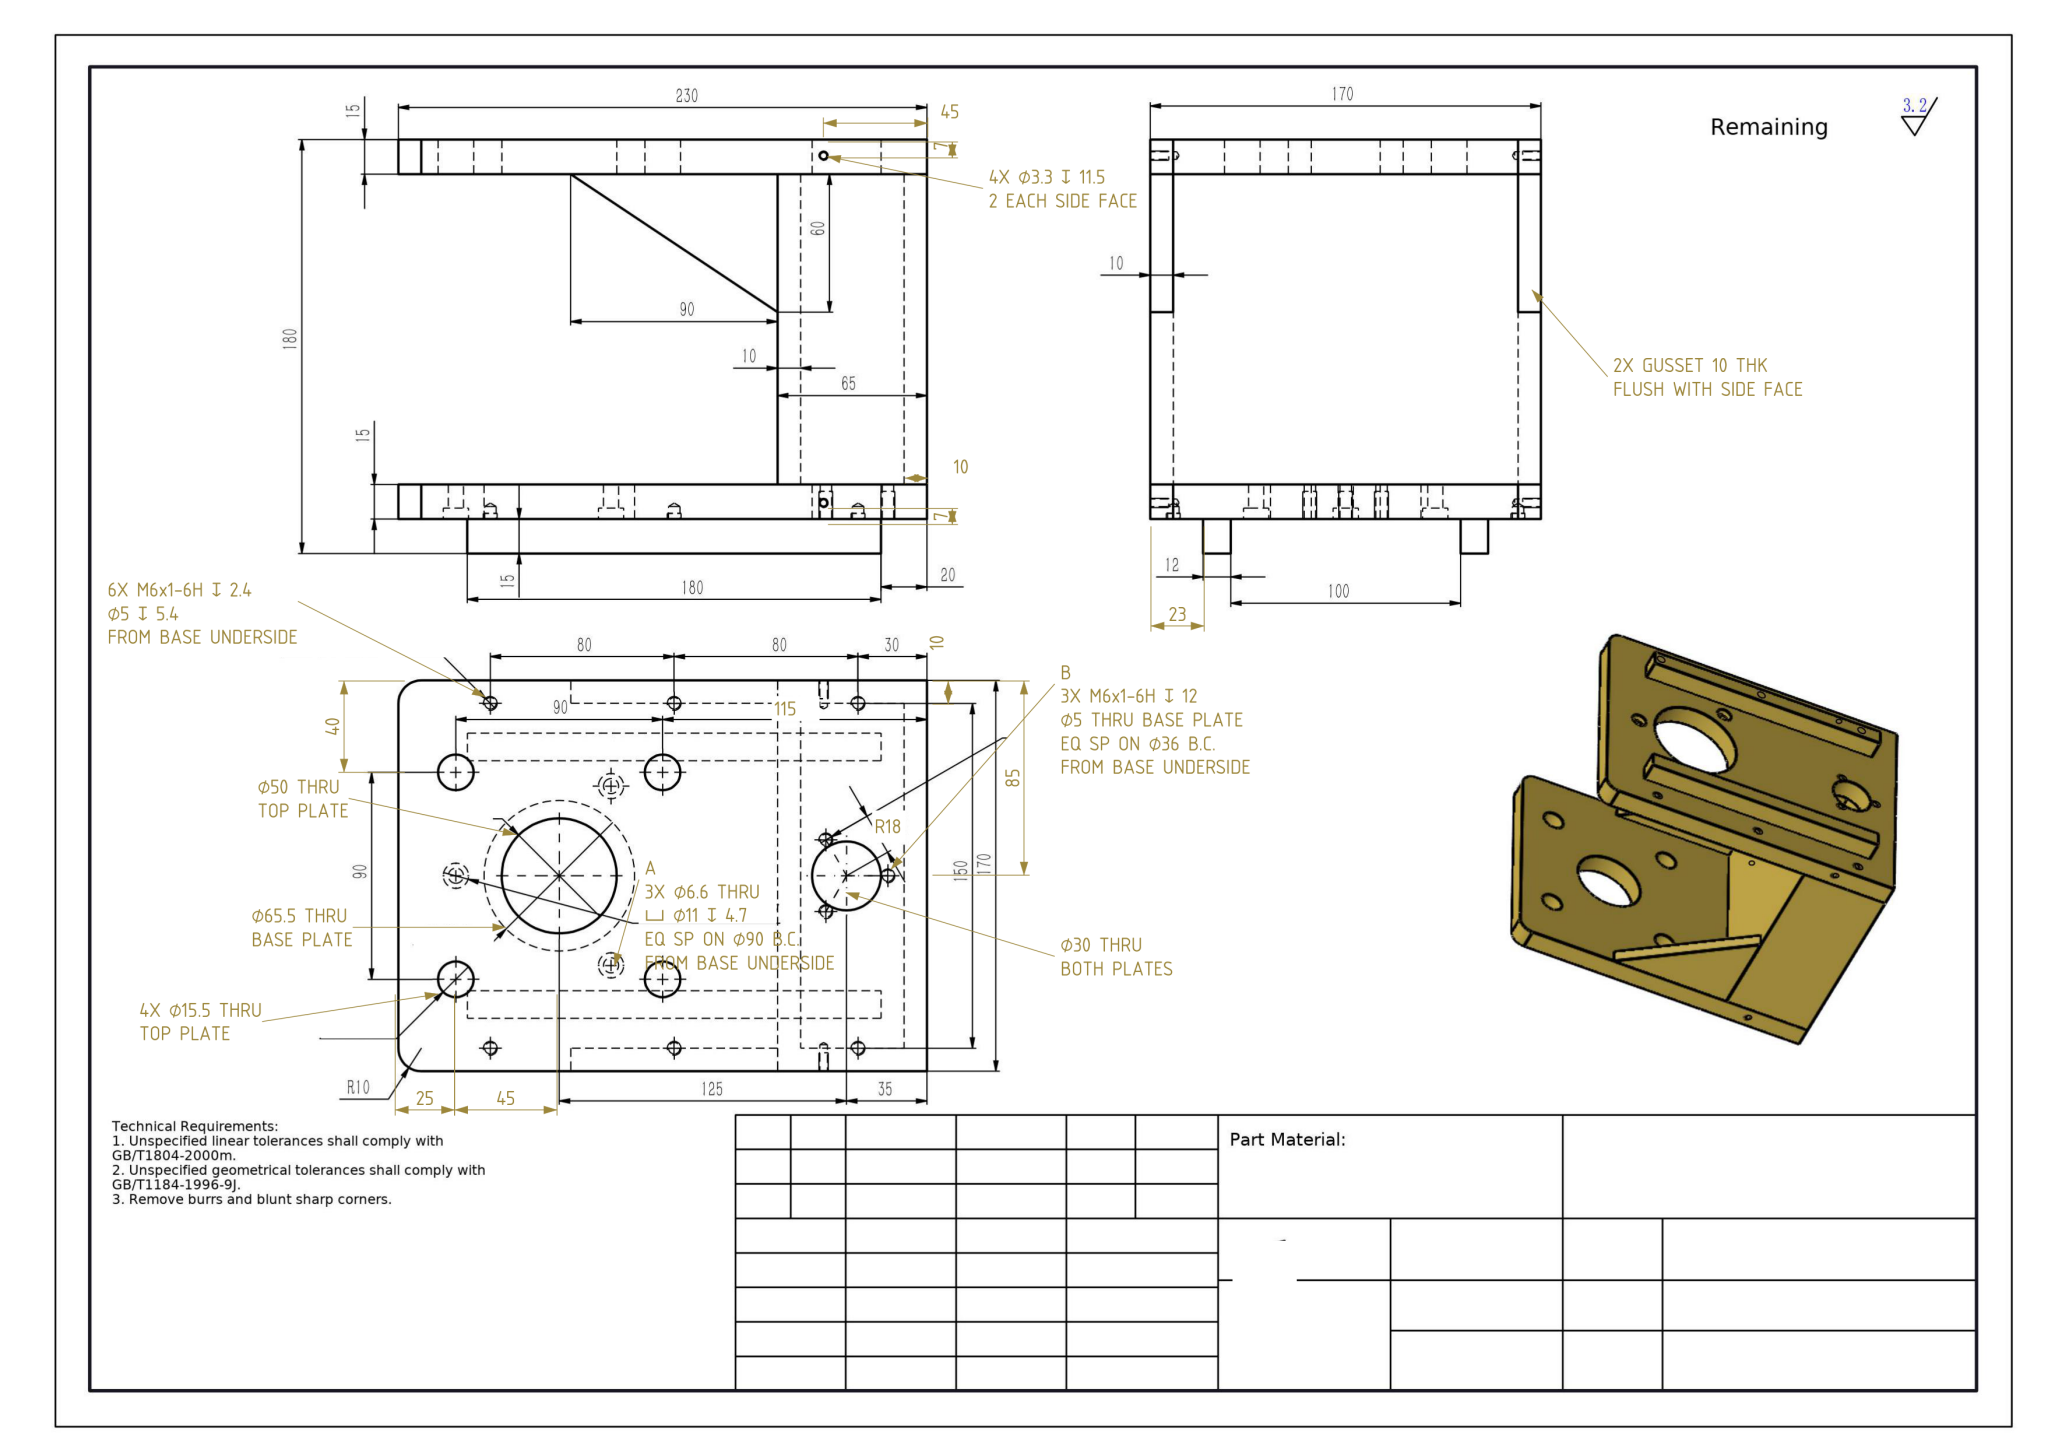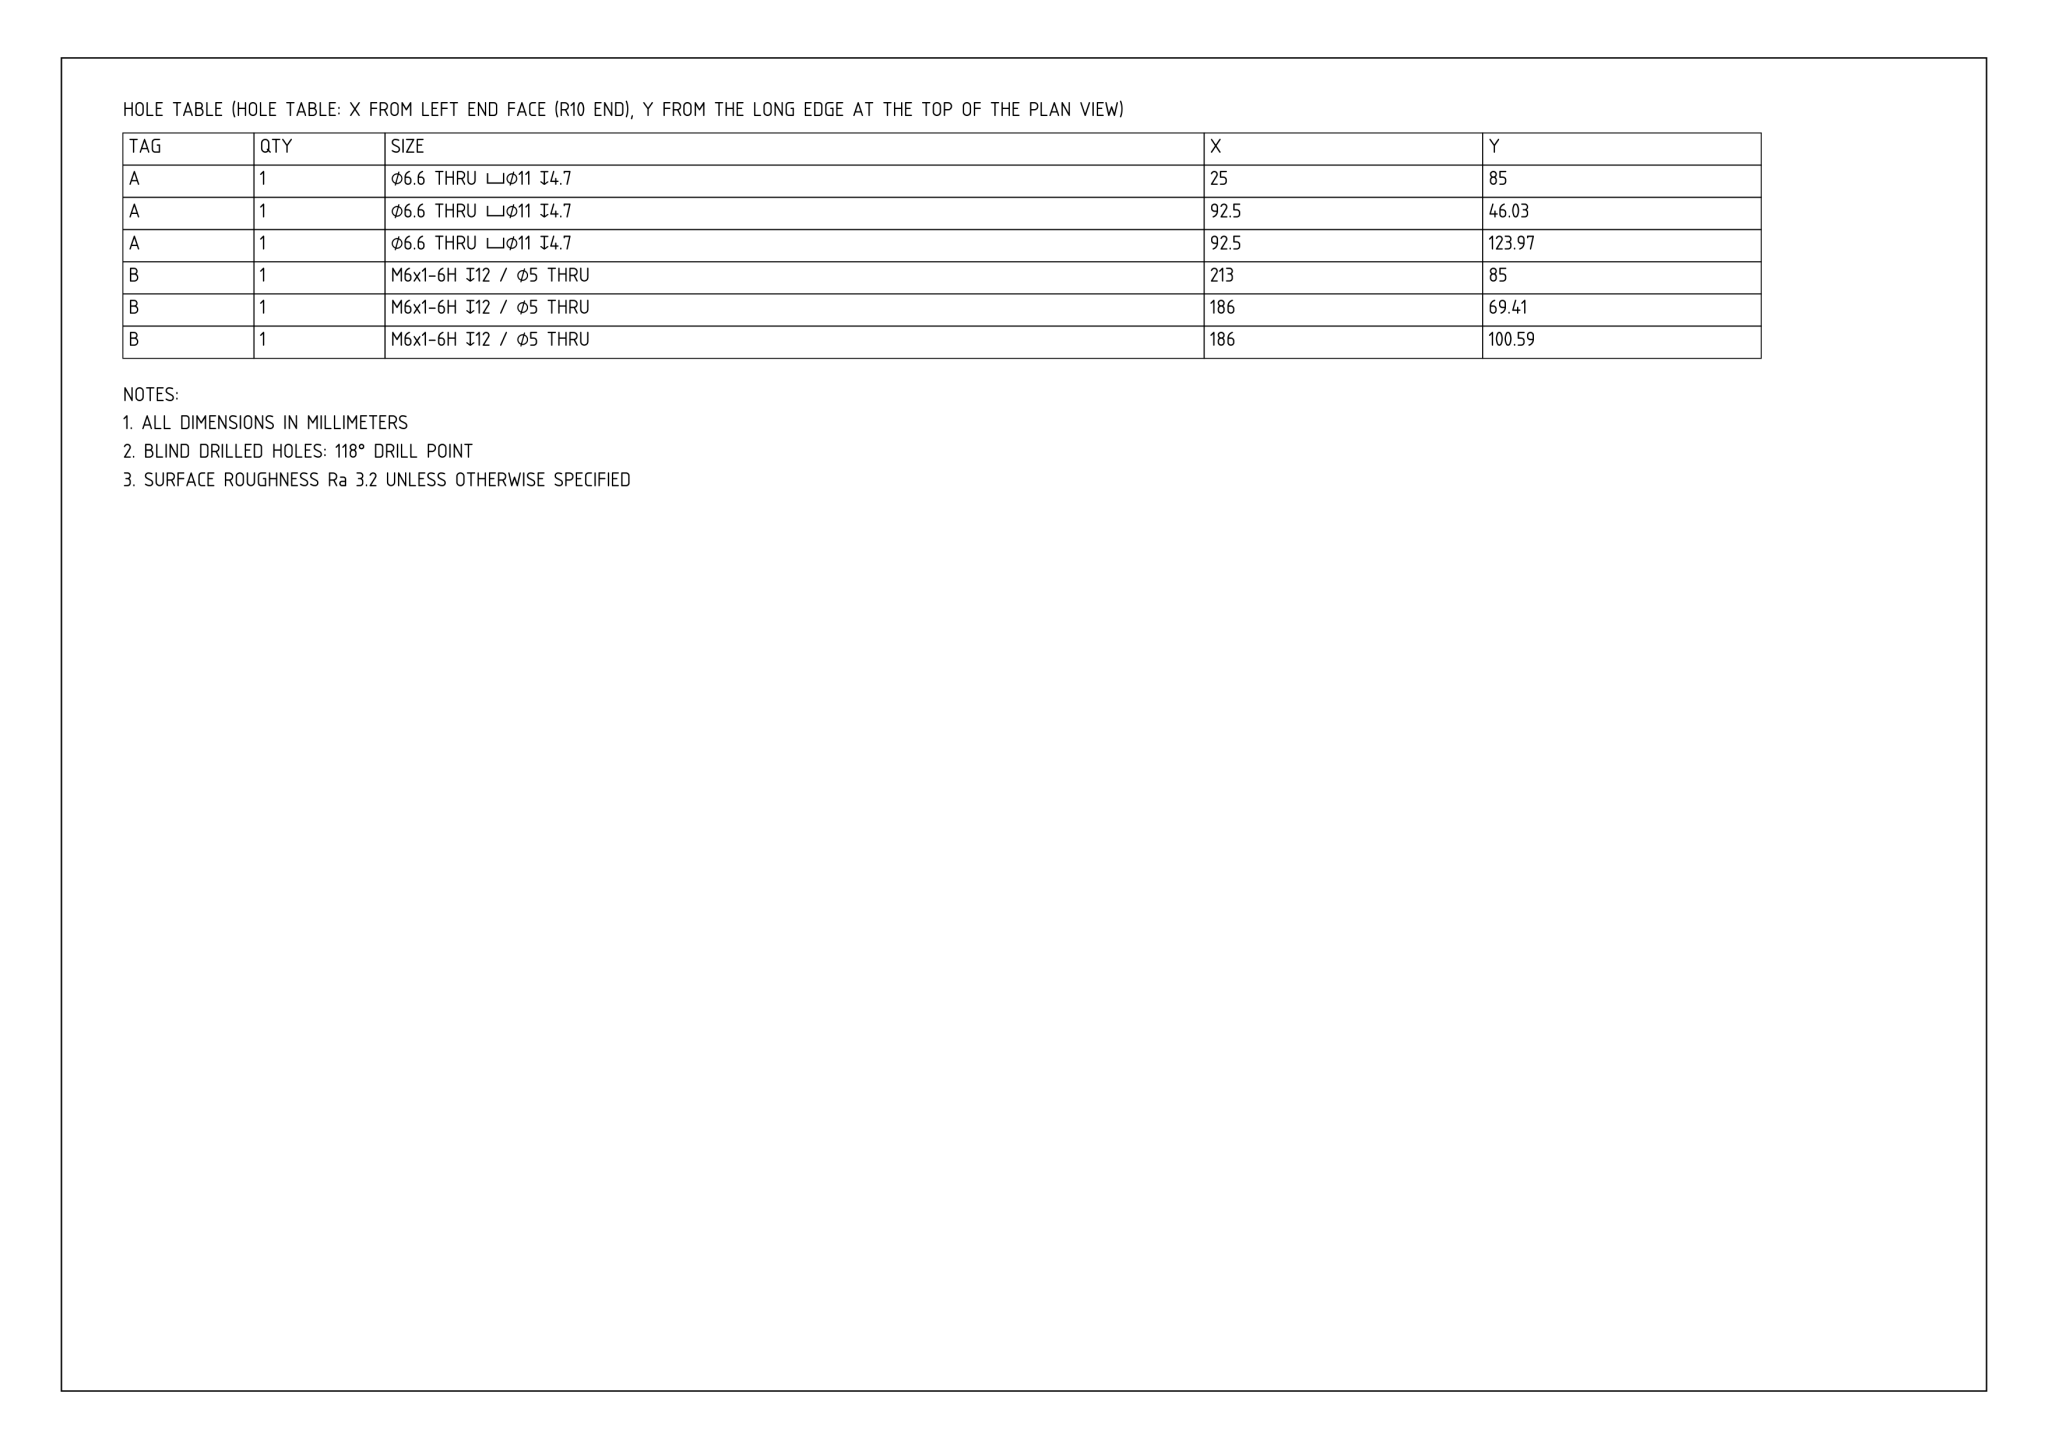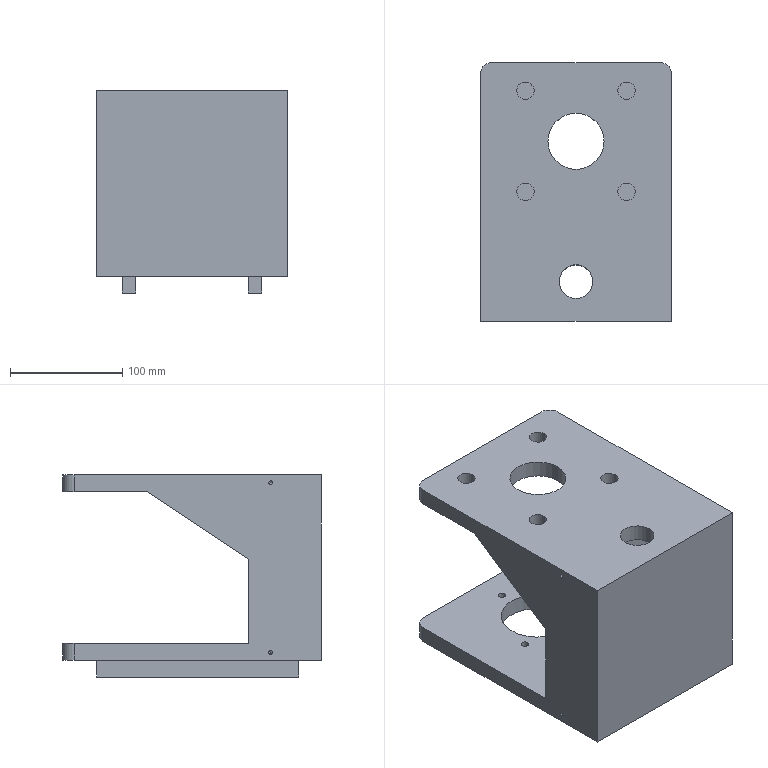Part | NX | mm | 1 solid | 111 faces | box 170 x 230 x 180 mm | volume 1754109 mm3 | cylinder 58 | plane 33 | cone 20 | commonest cylinder face diameters 5 x18 3.3 x8 15.5 x8 11 x6 6.6 x6 30 x4 20 x4 65.5 x2